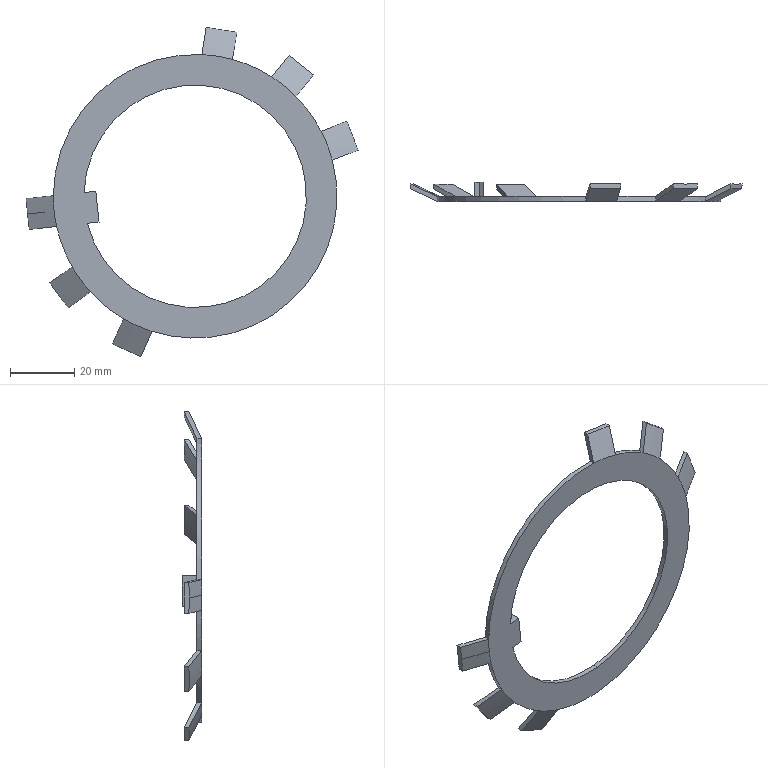Component | SolidWorks | LowerTensioningDeviceAssembly-1_GB858-1988[LockWasherForRoundNut68_1.5]-Driven2-1 | 1 solid | 49 faces | box 103.01 x 6 x 102.11 mm | volume 4358 mm3 | plane 25 | cone 14 | cylinder 10 | commonest cylinder face diameters 88 x7 69 x3
build123d program:
from build123d import *

# Parameters (mm, degrees)
SKETCH3_OUTSIDE_W   = 136.718
SKETCH3_OUTSIDE_H   = 136.718
CUT_EXTRUDE2_DEPTH  = 5.464
SKETCH4_W           = 9.6
SKETCH4_H           = 1.5
BOSS_EXTRUDE1_DEPTH = 6


with BuildPart() as part:
    # Sketch2 → Base-Revolve (revolve)
    with BuildSketch(Plane(origin=(0, 0, 0), x_dir=(0, 0, -1), z_dir=(1, 0, 0))):
        Polygon((-3.964, 52.5), (0, 44), (0, 0), (-1.5, 0), (-1.5, 44), (-5.464, 52.5), align=None)
    revolve(axis=Axis((0, 0, 0), (0, 0, 1)))

    # Sketch3 outside → Cut-Extrude2 (cut)
    # profile 1 of 2: a face of its own
    with BuildSketch(Plane.XY):
        Rectangle(SKETCH3_OUTSIDE_W, SKETCH3_OUTSIDE_H)
        with BuildLine():
            Line((-4.8, -43.737), (-4.8, -52.28))
            Line((-4.8, -52.28), (4.8, -52.28))
            Line((4.8, -52.28), (4.8, -43.737))
            ThreePointArc((4.8, -43.737), (34.908, -26.786), (43.489, 6.684))
            Line((43.489, 6.684), (51.741, 8.895))
            Line((51.741, 8.895), (49.256, 18.168))
            Line((49.256, 18.168), (41.005, 15.957))
            ThreePointArc((41.005, 15.957), (38.105, 22), (34.321, 27.533))
            Line((34.321, 27.533), (40.362, 33.574))
            Line((40.362, 33.574), (33.574, 40.362))
            Line((33.574, 40.362), (27.533, 34.321))
            ThreePointArc((27.533, 34.321), (22, 38.105), (15.957, 41.005))
            Line((15.957, 41.005), (18.168, 49.256))
            Line((18.168, 49.256), (8.895, 51.741))
            Line((8.895, 51.741), (6.684, 43.489))
            ThreePointArc((6.684, 43.489), (-34.908, 26.786), (-40.278, -17.712))
            Line((-40.278, -17.712), (-47.676, -21.983))
            Line((-47.676, -21.983), (-42.876, -30.297))
            Line((-42.876, -30.297), (-35.478, -26.026))
            ThreePointArc((-35.478, -26.026), (-31.113, -31.113), (-26.026, -35.478))
            Line((-26.026, -35.478), (-30.297, -42.876))
            Line((-30.297, -42.876), (-21.983, -47.676))
            Line((-21.983, -47.676), (-17.712, -40.278))
            ThreePointArc((-17.712, -40.278), (-11.388, -42.501), (-4.8, -43.737))
        make_face(mode=Mode.SUBTRACT)
    # profile 2 of 2: a face of its own
    with BuildSketch(Plane.XY):
        with BuildLine():
            Line((4.8, -34.164), (4.8, -30.5))
            Line((4.8, -30.5), (-4.8, -30.5))
            Line((-4.8, -30.5), (-4.8, -34.164))
            ThreePointArc((-4.8, -34.164), (0, 34.5), (4.8, -34.164))
        make_face()
    extrude(amount=CUT_EXTRUDE2_DEPTH, mode=Mode.SUBTRACT)

    # Sketch4 → Boss-Extrude1 (add)
    with BuildSketch(Plane.XY):
        with Locations((0, -31.25)):
            Rectangle(SKETCH4_W, SKETCH4_H)
    extrude(amount=BOSS_EXTRUDE1_DEPTH)


solid = part.part

# Placed as in the assembly
solid = solid.moved(Location((0, 180, -32.8), (-90, 0, -96.042)))